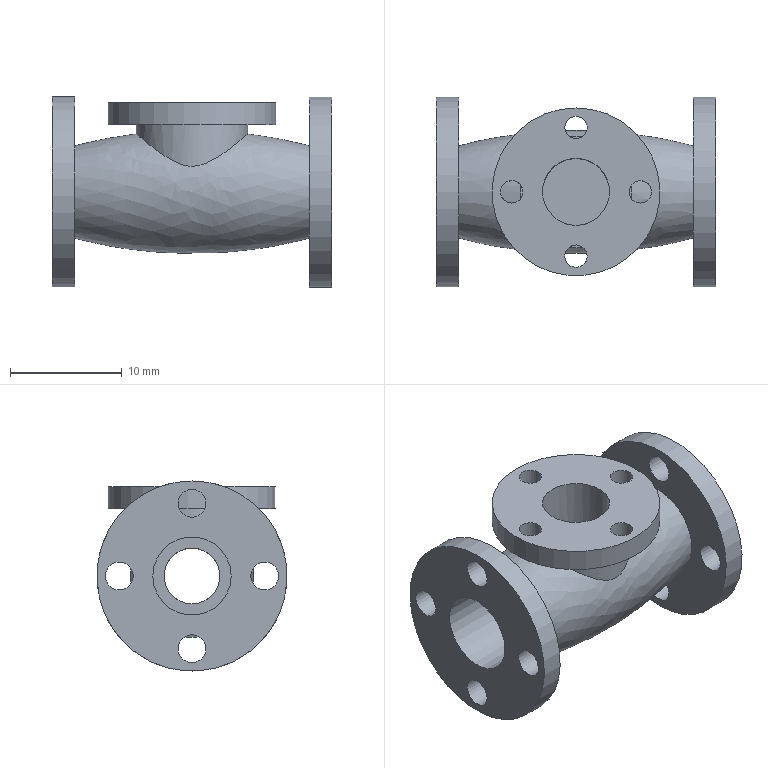Component | NX | EXT_PIPE | 1 solid | 35 faces | volume 2033 mm3 | cylinder 21 | plane 13 | spline 1 | commonest cylinder face diameters 2.5 x8 2 x4 17 x2 7 x2 5 x2 10 x1 15 x1 6 x1